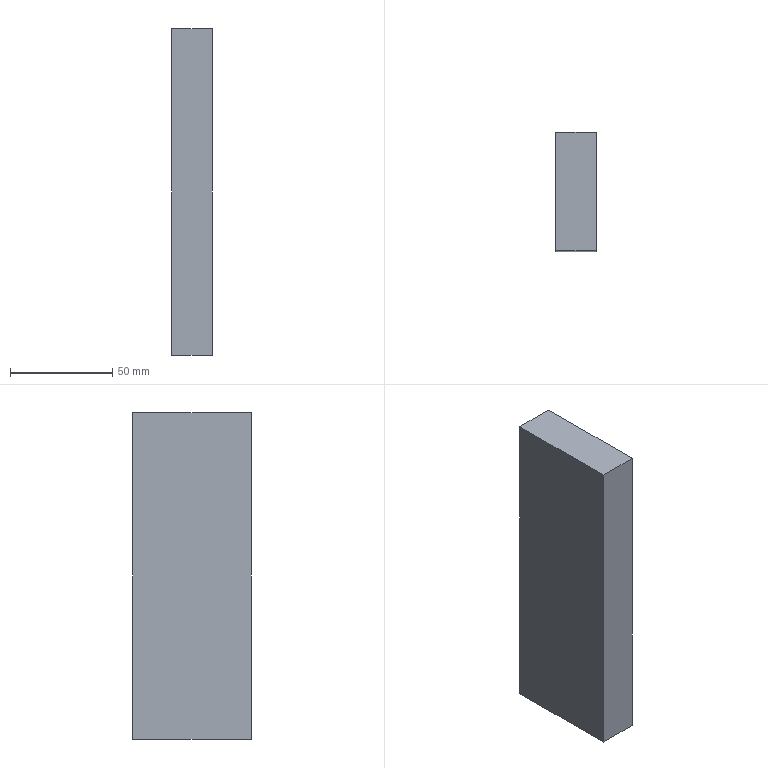Component | SolidWorks | Part18-1 | 1 solid | 6 faces | box 20 x 58 x 160 mm | volume 185600 mm3 | plane 6
build123d program:
from build123d import *

# Parameters (mm, degrees)
SKETCH1_W           = 160
SKETCH1_H           = 58
BOSS_EXTRUDE1_DEPTH = 20


with BuildPart() as part:
    # Sketch1 → Boss-Extrude1 (new body)
    with BuildSketch(Plane(origin=(0, 0, 0), x_dir=(0, 0, -1), z_dir=(1, 0, 0))):
        Rectangle(SKETCH1_W, SKETCH1_H)
    extrude(amount=BOSS_EXTRUDE1_DEPTH)


solid = part.part

# Placed as in the assembly
solid = solid.moved(Location((127.993, -512, -330), (0, 0, 0)))
STEP:
#1=CARTESIAN_POINT('',(5.039,-21.299,-16.142));
#2=VERTEX_POINT('',#1);
#3=CARTESIAN_POINT('',(5.039,-19.016,-16.142));
#4=VERTEX_POINT('',#3);
#5=CARTESIAN_POINT('',(5.039,-21.299,-16.142));
#6=DIRECTION('',(0.,1.,0.));
#7=VECTOR('',#6,39.37);
#8=LINE('',#5,#7);
#9=EDGE_CURVE('',#2,#4,#8,.T.);
#10=ORIENTED_EDGE('',*,*,#9,.T.);
#11=CARTESIAN_POINT('',(5.826,-19.016,-16.142));
#12=VERTEX_POINT('',#11);
#13=CARTESIAN_POINT('',(5.826,-19.016,-16.142));
#14=DIRECTION('',(-1.,0.,0.));
#15=VECTOR('',#14,39.37);
#16=LINE('',#13,#15);
#17=EDGE_CURVE('',#12,#4,#16,.T.);
#18=ORIENTED_EDGE('',*,*,#17,.F.);
#19=CARTESIAN_POINT('',(5.826,-21.299,-16.142));
#20=VERTEX_POINT('',#19);
#21=CARTESIAN_POINT('',(5.826,-21.299,-16.142));
#22=DIRECTION('',(0.,1.,0.));
#23=VECTOR('',#22,39.37);
#24=LINE('',#21,#23);
#25=EDGE_CURVE('',#20,#12,#24,.T.);
#26=ORIENTED_EDGE('',*,*,#25,.F.);
#27=CARTESIAN_POINT('',(5.826,-21.299,-16.142));
#28=DIRECTION('',(-1.,0.,0.));
#29=VECTOR('',#28,39.37);
#30=LINE('',#27,#29);
#31=EDGE_CURVE('',#20,#2,#30,.T.);
#32=ORIENTED_EDGE('',*,*,#31,.T.);
#33=EDGE_LOOP('',(#10,#18,#26,#32));
#34=FACE_OUTER_BOUND('',#33,.T.);
#35=CARTESIAN_POINT('',(5.826,-21.299,-16.142));
#36=DIRECTION('',(0.,0.,1.));
#37=DIRECTION('',(1.,0.,0.));
#38=AXIS2_PLACEMENT_3D('',#35,#36,#37);
#39=PLANE('',#38);
#40=ADVANCED_FACE('',(#34),#39,.F.);
#41=CARTESIAN_POINT('',(5.039,-19.016,-9.843));
#42=VERTEX_POINT('',#41);
#43=CARTESIAN_POINT('',(5.039,-19.016,-9.843));
#44=DIRECTION('',(0.,0.,1.));
#45=VECTOR('',#44,39.37);
#46=LINE('',#43,#45);
#47=EDGE_CURVE('',#4,#42,#46,.T.);
#48=ORIENTED_EDGE('',*,*,#47,.T.);
#49=CARTESIAN_POINT('',(5.826,-19.016,-9.843));
#50=VERTEX_POINT('',#49);
#51=CARTESIAN_POINT('',(5.826,-19.016,-9.843));
#52=DIRECTION('',(-1.,0.,0.));
#53=VECTOR('',#52,39.37);
#54=LINE('',#51,#53);
#55=EDGE_CURVE('',#50,#42,#54,.T.);
#56=ORIENTED_EDGE('',*,*,#55,.F.);
#57=CARTESIAN_POINT('',(5.826,-19.016,-9.843));
#58=DIRECTION('',(0.,0.,1.));
#59=VECTOR('',#58,39.37);
#60=LINE('',#57,#59);
#61=EDGE_CURVE('',#12,#50,#60,.T.);
#62=ORIENTED_EDGE('',*,*,#61,.F.);
#63=ORIENTED_EDGE('',*,*,#17,.T.);
#64=EDGE_LOOP('',(#48,#56,#62,#63));
#65=FACE_OUTER_BOUND('',#64,.T.);
#66=CARTESIAN_POINT('',(5.826,-19.016,-9.843));
#67=DIRECTION('',(0.,-1.,0.));
#68=DIRECTION('',(0.,0.,-1.));
#69=AXIS2_PLACEMENT_3D('',#66,#67,#68);
#70=PLANE('',#69);
#71=ADVANCED_FACE('',(#65),#70,.F.);
#72=CARTESIAN_POINT('',(5.039,-21.299,-9.843));
#73=VERTEX_POINT('',#72);
#74=CARTESIAN_POINT('',(5.039,-21.299,-9.843));
#75=DIRECTION('',(0.,-1.,0.));
#76=VECTOR('',#75,39.37);
#77=LINE('',#74,#76);
#78=EDGE_CURVE('',#42,#73,#77,.T.);
#79=ORIENTED_EDGE('',*,*,#78,.T.);
#80=CARTESIAN_POINT('',(5.826,-21.299,-9.843));
#81=VERTEX_POINT('',#80);
#82=CARTESIAN_POINT('',(5.826,-21.299,-9.843));
#83=DIRECTION('',(-1.,0.,0.));
#84=VECTOR('',#83,39.37);
#85=LINE('',#82,#84);
#86=EDGE_CURVE('',#81,#73,#85,.T.);
#87=ORIENTED_EDGE('',*,*,#86,.F.);
#88=CARTESIAN_POINT('',(5.826,-21.299,-9.843));
#89=DIRECTION('',(0.,-1.,0.));
#90=VECTOR('',#89,39.37);
#91=LINE('',#88,#90);
#92=EDGE_CURVE('',#50,#81,#91,.T.);
#93=ORIENTED_EDGE('',*,*,#92,.F.);
#94=ORIENTED_EDGE('',*,*,#55,.T.);
#95=EDGE_LOOP('',(#79,#87,#93,#94));
#96=FACE_OUTER_BOUND('',#95,.T.);
#97=CARTESIAN_POINT('',(5.826,-21.299,-9.843));
#98=DIRECTION('',(0.,0.,-1.));
#99=DIRECTION('',(-1.,0.,0.));
#100=AXIS2_PLACEMENT_3D('',#97,#98,#99);
#101=PLANE('',#100);
#102=ADVANCED_FACE('',(#96),#101,.F.);
#103=CARTESIAN_POINT('',(5.039,-21.299,-9.843));
#104=DIRECTION('',(0.,0.,-1.));
#105=VECTOR('',#104,39.37);
#106=LINE('',#103,#105);
#107=EDGE_CURVE('',#73,#2,#106,.T.);
#108=ORIENTED_EDGE('',*,*,#107,.T.);
#109=ORIENTED_EDGE('',*,*,#31,.F.);
#110=CARTESIAN_POINT('',(5.826,-21.299,-9.843));
#111=DIRECTION('',(0.,0.,-1.));
#112=VECTOR('',#111,39.37);
#113=LINE('',#110,#112);
#114=EDGE_CURVE('',#81,#20,#113,.T.);
#115=ORIENTED_EDGE('',*,*,#114,.F.);
#116=ORIENTED_EDGE('',*,*,#86,.T.);
#117=EDGE_LOOP('',(#108,#109,#115,#116));
#118=FACE_OUTER_BOUND('',#117,.T.);
#119=CARTESIAN_POINT('',(5.826,-21.299,-9.843));
#120=DIRECTION('',(0.,1.,0.));
#121=DIRECTION('',(0.,0.,1.));
#122=AXIS2_PLACEMENT_3D('',#119,#120,#121);
#123=PLANE('',#122);
#124=ADVANCED_FACE('',(#118),#123,.F.);
#125=ORIENTED_EDGE('',*,*,#25,.T.);
#126=ORIENTED_EDGE('',*,*,#61,.T.);
#127=ORIENTED_EDGE('',*,*,#92,.T.);
#128=ORIENTED_EDGE('',*,*,#114,.T.);
#129=EDGE_LOOP('',(#125,#126,#127,#128));
#130=FACE_OUTER_BOUND('',#129,.T.);
#131=CARTESIAN_POINT('',(5.826,-20.157,-12.992));
#132=DIRECTION('',(-1.,0.,0.));
#133=DIRECTION('',(0.,0.,1.));
#134=AXIS2_PLACEMENT_3D('',#131,#132,#133);
#135=PLANE('',#134);
#136=ADVANCED_FACE('',(#130),#135,.F.);
#137=ORIENTED_EDGE('',*,*,#9,.F.);
#138=ORIENTED_EDGE('',*,*,#107,.F.);
#139=ORIENTED_EDGE('',*,*,#78,.F.);
#140=ORIENTED_EDGE('',*,*,#47,.F.);
#141=EDGE_LOOP('',(#137,#138,#139,#140));
#142=FACE_OUTER_BOUND('',#141,.T.);
#143=CARTESIAN_POINT('',(5.039,-20.157,-12.992));
#144=DIRECTION('',(-1.,0.,0.));
#145=DIRECTION('',(0.,0.,1.));
#146=AXIS2_PLACEMENT_3D('',#143,#144,#145);
#147=PLANE('',#146);
#148=ADVANCED_FACE('',(#142),#147,.T.);
#149=CLOSED_SHELL('',(#40,#71,#102,#124,#136,#148));
#150=MANIFOLD_SOLID_BREP('',#149);
#151=CARTESIAN_POINT('',(0.,0.,0.));
#152=DIRECTION('',(0.,0.,1.));
#153=DIRECTION('',(1.,0.,0.));
#154=AXIS2_PLACEMENT_3D('',#151,#152,#153);
#155=(LENGTH_UNIT()NAMED_UNIT(*)SI_UNIT($,.METRE.));
#156=LENGTH_MEASURE_WITH_UNIT(LENGTH_MEASURE(0.0254),#155);
#157=DIMENSIONAL_EXPONENTS(1.,0.,0.,0.,0.,0.,0.);
#158=(CONVERSION_BASED_UNIT('',#156)LENGTH_UNIT()NAMED_UNIT(#157));
#159=UNCERTAINTY_MEASURE_WITH_UNIT(LENGTH_MEASURE(0.00001),#158,'','');
#160=(NAMED_UNIT(*)PLANE_ANGLE_UNIT()SI_UNIT($,.RADIAN.));
#161=(NAMED_UNIT(*)SI_UNIT($,.STERADIAN.)SOLID_ANGLE_UNIT());
#162=(GEOMETRIC_REPRESENTATION_CONTEXT(3)GLOBAL_UNCERTAINTY_ASSIGNED_CONTEXT((#159))GLOBAL_UNIT_ASSIGNED_CONTEXT((#158,#160,#161))REPRESENTATION_CONTEXT('',''));
#163=ADVANCED_BREP_SHAPE_REPRESENTATION('',(#150,#154),#162);
#164=COLOUR_RGB('',0.7922,0.8196,0.9333);
#165=FILL_AREA_STYLE_COLOUR('',#164);
#166=FILL_AREA_STYLE('',(#165));
#167=SURFACE_STYLE_FILL_AREA(#166);
#168=SURFACE_SIDE_STYLE('',(#167));
#169=SURFACE_STYLE_USAGE(.BOTH.,#168);
#170=PRESENTATION_STYLE_ASSIGNMENT((#169));
#171=STYLED_ITEM('',(#170),#150);
#172=PRESENTATION_LAYER_ASSIGNMENT('','',(#171));
#173=(LENGTH_UNIT()NAMED_UNIT(*)SI_UNIT($,.METRE.));
#174=LENGTH_MEASURE_WITH_UNIT(LENGTH_MEASURE(0.0254),#173);
#175=DIMENSIONAL_EXPONENTS(1.,0.,0.,0.,0.,0.,0.);
#176=(CONVERSION_BASED_UNIT('',#174)LENGTH_UNIT()NAMED_UNIT(#175));
#177=UNCERTAINTY_MEASURE_WITH_UNIT(LENGTH_MEASURE(0.00001),#176,'','');
#178=(NAMED_UNIT(*)PLANE_ANGLE_UNIT()SI_UNIT($,.RADIAN.));
#179=(NAMED_UNIT(*)SI_UNIT($,.STERADIAN.)SOLID_ANGLE_UNIT());
#180=(GEOMETRIC_REPRESENTATION_CONTEXT(3)GLOBAL_UNCERTAINTY_ASSIGNED_CONTEXT((#177))GLOBAL_UNIT_ASSIGNED_CONTEXT((#176,#178,#179))REPRESENTATION_CONTEXT('',''));
#181=MECHANICAL_DESIGN_GEOMETRIC_PRESENTATION_REPRESENTATION('',(#171),#180);